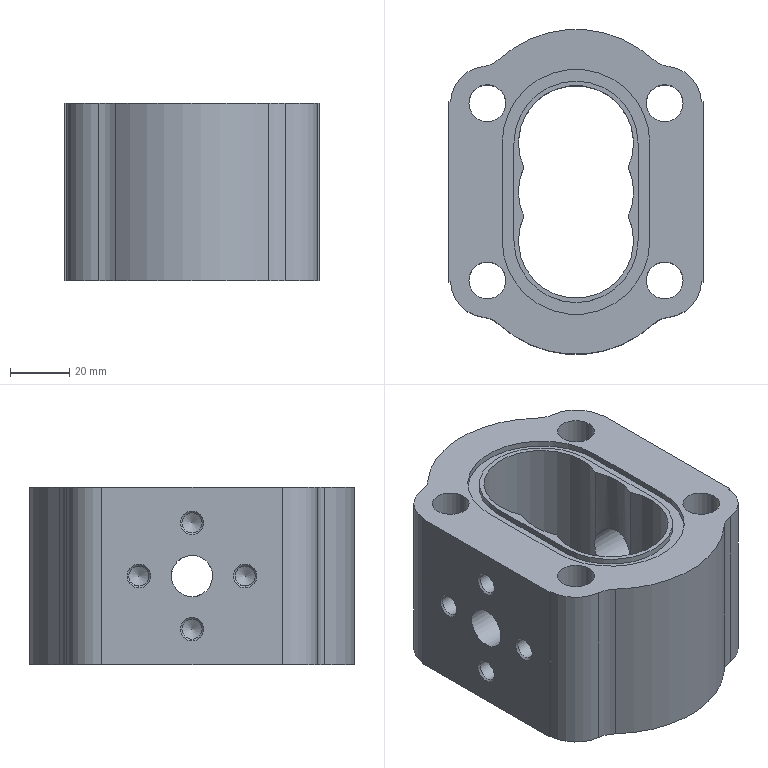Component | NX | 2 | 1 solid | 77 faces | volume 292855 mm3 | cylinder 39 | plane 20 | cone 18 | commonest cylinder face diameters 6.8 x8 39 x5 25 x4 20 x4 12.5 x4 42 x4 50 x4 77 x2